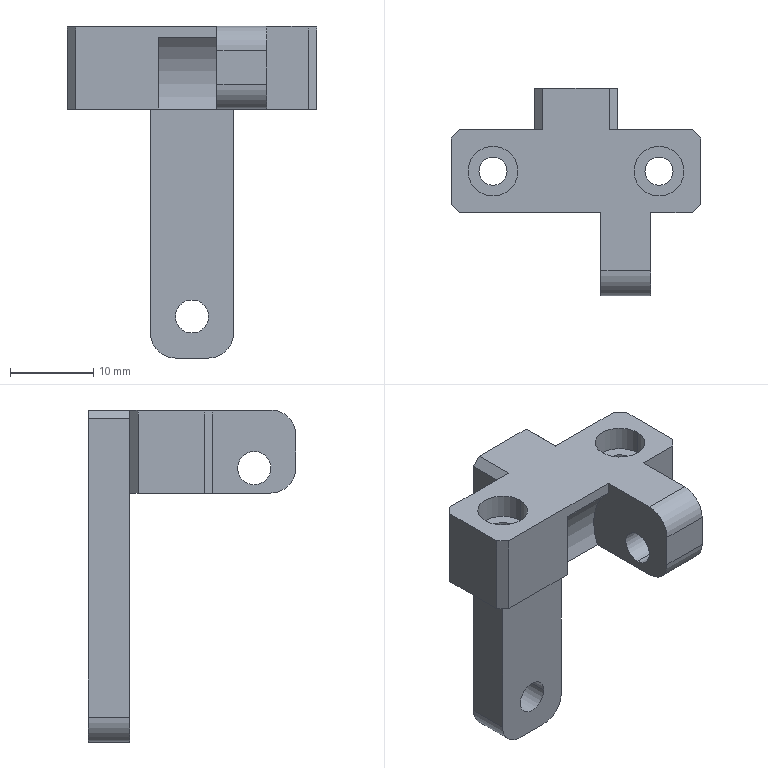Component | SolidWorks | WZH-20190520-F212StopBlockPusher-1 | 1 solid | 48 faces | box 30 x 25 x 40 mm | volume 4838 mm3 | plane 27 | cylinder 21 | commonest cylinder face diameters 6 x8 6.2 x4 4 x4 3.4 x4 15 x1 | material 45
build123d program:
from build123d import *

# Parameters (mm, degrees)
SKETCH2_W           = 10
SKETCH2_H           = 30
BOSS_EXTRUDE1_DEPTH = 5
SKETCH3_W           = 40
SKETCH3_H           = 10
BOSS_EXTRUDE2_DEPTH = 5
SKETCH4_R           = 3
CUT_EXTRUDE1_DEPTH  = 3
SKETCH5_R           = 1.7
CUT_EXTRUDE2_DEPTH  = 42.158
SKETCH6_W           = 10
SKETCH6_H           = 6
BOSS_EXTRUDE3_DEPTH = 10
M4_TAPPED_HOLE1_D   = 4
M4_TAPPED_HOLE2_D   = 4
SKETCH11_R          = 7.5
CUT_EXTRUDE3_DEPTH  = 7
FILLET1_R           = 3
CHAMFER1_SIZE       = 1
SKETCH12_R          = 3.1
CUT_EXTRUDE4_DEPTH  = 3.4


with BuildPart() as part:
    # Sketch2 → Boss-Extrude1 (new, symmetric)
    with BuildSketch(Plane(origin=(0, 0, 0), x_dir=(1, 0, 0), z_dir=(0, 1, 0))):
        Rectangle(SKETCH2_W, SKETCH2_H)
    extrude(amount=BOSS_EXTRUDE1_DEPTH, both=True)

    # Sketch3 → Boss-Extrude2 (add)
    with BuildSketch(Plane(origin=(0, 5, 0), x_dir=(1, 0, 0), z_dir=(0, 1, 0))):
        with Locations((-15, 0)):
            Rectangle(SKETCH3_W, SKETCH3_H)
    extrude(amount=BOSS_EXTRUDE2_DEPTH)

    # Sketch4 → Cut-Extrude1 (cut)
    with BuildSketch(Plane(origin=(5, 0, 0), x_dir=(0, 0, -1), z_dir=(1, 0, 0))):
        with Locations((-10, 0)):
            Circle(SKETCH4_R)
        with Locations((10, 0)):
            Circle(SKETCH4_R)
    extrude(amount=-CUT_EXTRUDE1_DEPTH, mode=Mode.SUBTRACT)

    # Sketch5 → Cut-Extrude2 (cut, through all)
    with BuildSketch(Plane(origin=(2, 0, 0), x_dir=(0, 0, -1), z_dir=(1, 0, 0))):
        with Locations((10, 0)):
            Circle(SKETCH5_R)
        with Locations((-10, 0)):
            Circle(SKETCH5_R)
    extrude(amount=-CUT_EXTRUDE2_DEPTH, mode=Mode.SUBTRACT)

    # Sketch6 → Boss-Extrude3 (add)
    with BuildSketch(Plane.XZ.offset(5)):
        with Locations((0, -6)):
            Rectangle(SKETCH6_W, SKETCH6_H)
    extrude(amount=BOSS_EXTRUDE3_DEPTH)

    # M4 Tapped Hole1 (through all)
    with Locations(Plane.XY.offset(-3)):
        with Locations((-2, -10)):
            Hole(M4_TAPPED_HOLE1_D / 2)

    # M4 Tapped Hole2 (through all)
    with Locations(Plane(origin=(0, 10, 0), x_dir=(1, 0, 0), z_dir=(0, 1, 0))):
        with Locations((-30, 0)):
            Hole(M4_TAPPED_HOLE2_D / 2)

    # Sketch11 → Cut-Extrude3 (cut)
    with BuildSketch(Plane.XY.offset(-3)):
        with Locations((-2, -10)):
            Circle(SKETCH11_R)
    extrude(amount=CUT_EXTRUDE3_DEPTH, mode=Mode.SUBTRACT)

    # Fillet1
    fillet1_edges = [part.edges().sort_by_distance(p)[0] for p in [
        (-35, 7.5, -5),
        (-35, 7.5, 5),
        (-5, -15, -6),
        (5, -15, -6),
    ]]
    fillet(fillet1_edges, radius=FILLET1_R)

    # Chamfer1
    chamfer1_edges = [part.edges().sort_by_distance(p)[0] for p in [
        (0, 5, -15),
        (5, 7.5, 5),
        (5, 7.5, -5),
        (0, -5, -15),
        (0, -5, 15),
        (0, 5, 15),
    ]]
    chamfer(chamfer1_edges, length=CHAMFER1_SIZE)

    # Sketch12 → Cut-Extrude4 (cut)
    with BuildSketch(Plane.ZY.offset(5)):
        with Locations((10, 0)):
            Circle(SKETCH12_R)
        with Locations((-10, 0)):
            Circle(SKETCH12_R)
    extrude(amount=-CUT_EXTRUDE4_DEPTH, mode=Mode.SUBTRACT)


solid = part.part

# Placed as in the assembly
solid = solid.moved(Location((0, 5.5, -25.446), (0, -90, 0)))